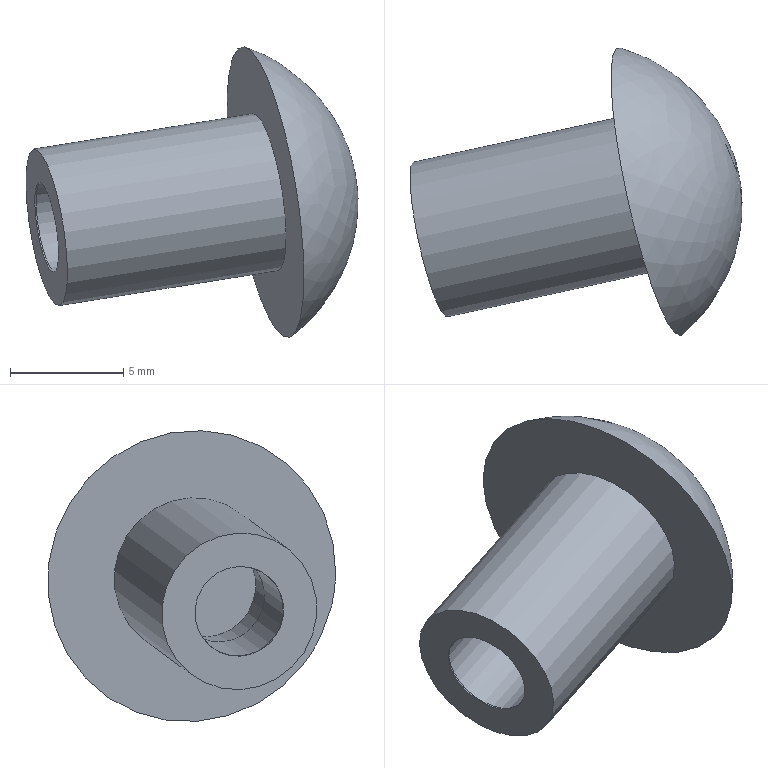Component | NX | 1_10 | 1 solid | 9 faces | box 14.65 x 12.71 x 12.84 mm | volume 581 mm3 | plane 4 | cylinder 3 | cone 1 | spline 1 | commonest cylinder face diameters 7 x1 4 x1 4.5 x1
STEP:
#1=CARTESIAN_POINT('',(0.,0.,0.));
#2=DIRECTION('',(0.,0.,1.));
#3=DIRECTION('',(1.,0.,0.));
#4=AXIS2_PLACEMENT_3D('',#1,#2,#3);
#5=CARTESIAN_POINT('',(119.694,214.706,-143.655));
#6=VERTEX_POINT('',#5);
#7=CARTESIAN_POINT('',(120.69,211.014,-144.855));
#8=VERTEX_POINT('',#7);
#9=CARTESIAN_POINT('',(120.192,212.86,-144.255));
#10=DIRECTION('',(0.9653,0.21,0.1554));
#11=DIRECTION('',(-0.2486,0.9212,0.2993));
#12=AXIS2_PLACEMENT_3D('',#9,#10,#11);
#13=CIRCLE('',#12,2.004);
#14=CARTESIAN_POINT('',(121.062,209.636,-145.303));
#15=DIRECTION('',(-0.9653,-0.21,-0.1554));
#16=DIRECTION('',(0.2486,-0.9212,-0.2993));
#17=AXIS2_PLACEMENT_3D('',#14,#15,#16);
#18=PLANE('',#17);
#19=CARTESIAN_POINT('',(-5.504,0.));
#20=CARTESIAN_POINT('',(-5.504,3.471));
#21=CARTESIAN_POINT('',(-2.498,1.735));
#22=CARTESIAN_POINT('',(0.5078,0.));
#23=CARTESIAN_POINT('',(-2.498,-1.735));
#24=CARTESIAN_POINT('',(-5.504,-3.471));
#25=CARTESIAN_POINT('',(-5.504,0.));
#26=(BOUNDED_CURVE()B_SPLINE_CURVE(2,(#19,#20,#21,#22,#23,#24,#25),.UNSPECIFIED.,.T.,.F.)B_SPLINE_CURVE_WITH_KNOTS((1,2,2,2,2,1),(-2.094,0.,2.094,4.189,6.283,8.378),.UNSPECIFIED.)CURVE()GEOMETRIC_REPRESENTATION_ITEM()RATIONAL_B_SPLINE_CURVE((1.,0.5,1.,0.5,1.,0.5,1.))REPRESENTATION_ITEM(''));
#27=(GEOMETRIC_REPRESENTATION_CONTEXT(2)PARAMETRIC_REPRESENTATION_CONTEXT()REPRESENTATION_CONTEXT('',''));
#28=DEFINITIONAL_REPRESENTATION('',(#26),#27);
#29=PCURVE('',#18,#28);
#30=CARTESIAN_POINT('',(120.192,212.86,-144.255));
#31=DIRECTION('',(-0.9653,-0.21,-0.1554));
#32=DIRECTION('',(0.2486,-0.9212,-0.2993));
#33=AXIS2_PLACEMENT_3D('',#30,#31,#32);
#34=CONICAL_SURFACE('',#33,2.004,0.0629);
#35=CARTESIAN_POINT('',(3.142,0.));
#36=DIRECTION('',(-1.,0.));
#37=VECTOR('',#36,1.);
#38=LINE('',#35,#37);
#39=(GEOMETRIC_REPRESENTATION_CONTEXT(2)PARAMETRIC_REPRESENTATION_CONTEXT()REPRESENTATION_CONTEXT('',''));
#40=DEFINITIONAL_REPRESENTATION('',(#38),#39);
#41=PCURVE('',#34,#40);
#42=SURFACE_CURVE('',#13,(#29,#41),.PCURVE_S1.);
#43=EDGE_CURVE('',#6,#8,#42,.T.);
#44=ORIENTED_EDGE('',*,*,#43,.T.);
#45=CARTESIAN_POINT('',(120.192,212.86,-144.255));
#46=DIRECTION('',(0.9653,0.21,0.1554));
#47=DIRECTION('',(-0.2486,0.9212,0.2993));
#48=AXIS2_PLACEMENT_3D('',#45,#46,#47);
#49=CIRCLE('',#48,2.004);
#50=CARTESIAN_POINT('',(-5.504,0.));
#51=CARTESIAN_POINT('',(-5.504,3.471));
#52=CARTESIAN_POINT('',(-2.498,1.735));
#53=CARTESIAN_POINT('',(0.5078,0.));
#54=CARTESIAN_POINT('',(-2.498,-1.735));
#55=CARTESIAN_POINT('',(-5.504,-3.471));
#56=CARTESIAN_POINT('',(-5.504,0.));
#57=(BOUNDED_CURVE()B_SPLINE_CURVE(2,(#50,#51,#52,#53,#54,#55,#56),.UNSPECIFIED.,.T.,.F.)B_SPLINE_CURVE_WITH_KNOTS((1,2,2,2,2,1),(-2.094,0.,2.094,4.189,6.283,8.378),.UNSPECIFIED.)CURVE()GEOMETRIC_REPRESENTATION_ITEM()RATIONAL_B_SPLINE_CURVE((1.,0.5,1.,0.5,1.,0.5,1.))REPRESENTATION_ITEM(''));
#58=(GEOMETRIC_REPRESENTATION_CONTEXT(2)PARAMETRIC_REPRESENTATION_CONTEXT()REPRESENTATION_CONTEXT('',''));
#59=DEFINITIONAL_REPRESENTATION('',(#57),#58);
#60=PCURVE('',#18,#59);
#61=CARTESIAN_POINT('',(9.425,0.));
#62=DIRECTION('',(-1.,0.));
#63=VECTOR('',#62,1.);
#64=LINE('',#61,#63);
#65=(GEOMETRIC_REPRESENTATION_CONTEXT(2)PARAMETRIC_REPRESENTATION_CONTEXT()REPRESENTATION_CONTEXT('',''));
#66=DEFINITIONAL_REPRESENTATION('',(#64),#65);
#67=PCURVE('',#34,#66);
#68=SURFACE_CURVE('',#49,(#60,#67),.PCURVE_S1.);
#69=EDGE_CURVE('',#8,#6,#68,.T.);
#70=ORIENTED_EDGE('',*,*,#69,.T.);
#71=EDGE_LOOP('',(#44,#70));
#72=FACE_BOUND('',#71,.T.);
#73=CARTESIAN_POINT('',(119.322,216.084,-143.208));
#74=VERTEX_POINT('',#73);
#75=CARTESIAN_POINT('',(120.192,212.86,-144.255));
#76=DIRECTION('',(0.9653,0.21,0.1554));
#77=DIRECTION('',(-0.2486,0.9212,0.2993));
#78=AXIS2_PLACEMENT_3D('',#75,#76,#77);
#79=CIRCLE('',#78,3.5);
#80=CARTESIAN_POINT('',(-7.,0.));
#81=CARTESIAN_POINT('',(-7.,6.062));
#82=CARTESIAN_POINT('',(-1.75,3.031));
#83=CARTESIAN_POINT('',(3.5,0.));
#84=CARTESIAN_POINT('',(-1.75,-3.031));
#85=CARTESIAN_POINT('',(-7.,-6.062));
#86=CARTESIAN_POINT('',(-7.,0.));
#87=(BOUNDED_CURVE()B_SPLINE_CURVE(2,(#80,#81,#82,#83,#84,#85,#86),.UNSPECIFIED.,.T.,.F.)B_SPLINE_CURVE_WITH_KNOTS((1,2,2,2,2,1),(-2.094,0.,2.094,4.189,6.283,8.378),.UNSPECIFIED.)CURVE()GEOMETRIC_REPRESENTATION_ITEM()RATIONAL_B_SPLINE_CURVE((1.,0.5,1.,0.5,1.,0.5,1.))REPRESENTATION_ITEM(''));
#88=(GEOMETRIC_REPRESENTATION_CONTEXT(2)PARAMETRIC_REPRESENTATION_CONTEXT()REPRESENTATION_CONTEXT('',''));
#89=DEFINITIONAL_REPRESENTATION('',(#87),#88);
#90=PCURVE('',#18,#89);
#91=CARTESIAN_POINT('',(129.845,214.96,-142.701));
#92=DIRECTION('',(0.9653,0.21,0.1554));
#93=DIRECTION('',(-0.2486,0.9212,0.2993));
#94=AXIS2_PLACEMENT_3D('',#91,#92,#93);
#95=CYLINDRICAL_SURFACE('',#94,3.5);
#96=CARTESIAN_POINT('',(0.,-10.));
#97=DIRECTION('',(1.,0.));
#98=VECTOR('',#97,1.);
#99=LINE('',#96,#98);
#100=(GEOMETRIC_REPRESENTATION_CONTEXT(2)PARAMETRIC_REPRESENTATION_CONTEXT()REPRESENTATION_CONTEXT('',''));
#101=DEFINITIONAL_REPRESENTATION('',(#99),#100);
#102=PCURVE('',#95,#101);
#103=SURFACE_CURVE('',#79,(#90,#102),.PCURVE_S1.);
#104=EDGE_CURVE('',#74,#74,#103,.T.);
#105=ORIENTED_EDGE('',*,*,#104,.F.);
#106=EDGE_LOOP('',(#105));
#107=FACE_BOUND('',#106,.T.);
#108=ADVANCED_FACE('',(#72,#107),#18,.T.);
#109=CARTESIAN_POINT('',(120.749,211.03,-144.844));
#110=VERTEX_POINT('',#109);
#111=CARTESIAN_POINT('',(120.252,212.873,-144.246));
#112=DIRECTION('',(-0.9653,-0.21,-0.1554));
#113=DIRECTION('',(0.2486,-0.9212,-0.2993));
#114=AXIS2_PLACEMENT_3D('',#111,#112,#113);
#115=CIRCLE('',#114,2.);
#116=CARTESIAN_POINT('',(0.,-0.06178));
#117=DIRECTION('',(1.,0.));
#118=VECTOR('',#117,1.);
#119=LINE('',#116,#118);
#120=(GEOMETRIC_REPRESENTATION_CONTEXT(2)PARAMETRIC_REPRESENTATION_CONTEXT()REPRESENTATION_CONTEXT('',''));
#121=DEFINITIONAL_REPRESENTATION('',(#119),#120);
#122=PCURVE('',#34,#121);
#123=CARTESIAN_POINT('',(124.053,213.7,-143.633));
#124=DIRECTION('',(-0.9653,-0.21,-0.1554));
#125=DIRECTION('',(0.2486,-0.9212,-0.2993));
#126=AXIS2_PLACEMENT_3D('',#123,#124,#125);
#127=CYLINDRICAL_SURFACE('',#126,2.);
#128=CARTESIAN_POINT('',(0.,3.938));
#129=DIRECTION('',(1.,0.));
#130=VECTOR('',#129,1.);
#131=LINE('',#128,#130);
#132=(GEOMETRIC_REPRESENTATION_CONTEXT(2)PARAMETRIC_REPRESENTATION_CONTEXT()REPRESENTATION_CONTEXT('',''));
#133=DEFINITIONAL_REPRESENTATION('',(#131),#132);
#134=PCURVE('',#127,#133);
#135=SURFACE_CURVE('',#115,(#122,#134),.PCURVE_S1.);
#136=EDGE_CURVE('',#110,#110,#135,.T.);
#137=ORIENTED_EDGE('',*,*,#136,.T.);
#138=CARTESIAN_POINT('',(120.749,211.03,-144.844));
#139=CARTESIAN_POINT('',(120.69,211.014,-144.855));
#140=B_SPLINE_CURVE_WITH_KNOTS('',1,(#138,#139),.UNSPECIFIED.,.F.,.F.,(2,2),(-0.0619,0.),.PIECEWISE_BEZIER_KNOTS.);
#141=CARTESIAN_POINT('',(6.283,0.));
#142=DIRECTION('',(0.,1.));
#143=VECTOR('',#142,1.);
#144=LINE('',#141,#143);
#145=(GEOMETRIC_REPRESENTATION_CONTEXT(2)PARAMETRIC_REPRESENTATION_CONTEXT()REPRESENTATION_CONTEXT('',''));
#146=DEFINITIONAL_REPRESENTATION('',(#144),#145);
#147=PCURVE('',#34,#146);
#148=CARTESIAN_POINT('',(0.,0.));
#149=DIRECTION('',(0.,1.));
#150=VECTOR('',#149,1.);
#151=LINE('',#148,#150);
#152=(GEOMETRIC_REPRESENTATION_CONTEXT(2)PARAMETRIC_REPRESENTATION_CONTEXT()REPRESENTATION_CONTEXT('',''));
#153=DEFINITIONAL_REPRESENTATION('',(#151),#152);
#154=PCURVE('',#34,#153);
#155=SEAM_CURVE('',#140,(#147,#154),.PCURVE_S1.);
#156=EDGE_CURVE('',#110,#8,#155,.T.);
#157=ORIENTED_EDGE('',*,*,#156,.T.);
#158=ORIENTED_EDGE('',*,*,#69,.T.);
#159=ORIENTED_EDGE('',*,*,#43,.T.);
#160=ORIENTED_EDGE('',*,*,#156,.F.);
#161=EDGE_LOOP('',(#137,#157,#158,#159,#160));
#162=FACE_BOUND('',#161,.F.);
#163=ADVANCED_FACE('',(#162),#34,.F.);
#164=CARTESIAN_POINT('',(128.229,220.948,-140.755));
#165=VERTEX_POINT('',#164);
#166=CARTESIAN_POINT('',(129.845,214.96,-142.701));
#167=DIRECTION('',(0.9653,0.21,0.1554));
#168=DIRECTION('',(-0.2486,0.9212,0.2993));
#169=AXIS2_PLACEMENT_3D('',#166,#167,#168);
#170=CIRCLE('',#169,6.5);
#171=CARTESIAN_POINT('',(133.706,215.8,-142.079));
#172=CARTESIAN_POINT('',(133.706,215.8,-142.079));
#173=CARTESIAN_POINT('',(133.706,215.8,-142.079));
#174=CARTESIAN_POINT('',(133.706,215.8,-142.079));
#175=CARTESIAN_POINT('',(133.706,215.8,-142.079));
#176=CARTESIAN_POINT('',(133.706,215.8,-142.079));
#177=CARTESIAN_POINT('',(133.706,215.8,-142.079));
#178=CARTESIAN_POINT('',(132.96,218.372,-141.248));
#179=CARTESIAN_POINT('',(132.51,216.535,-135.969));
#180=CARTESIAN_POINT('',(133.904,211.37,-137.647));
#181=CARTESIAN_POINT('',(134.354,213.207,-142.926));
#182=CARTESIAN_POINT('',(134.805,215.043,-148.205));
#183=CARTESIAN_POINT('',(133.411,220.209,-146.527));
#184=CARTESIAN_POINT('',(132.96,218.372,-141.248));
#185=CARTESIAN_POINT('',(130.948,220.263,-140.761));
#186=CARTESIAN_POINT('',(130.114,216.862,-130.986));
#187=CARTESIAN_POINT('',(132.695,207.297,-134.094));
#188=CARTESIAN_POINT('',(133.53,210.698,-143.869));
#189=CARTESIAN_POINT('',(134.364,214.099,-153.645));
#190=CARTESIAN_POINT('',(131.782,223.665,-150.537));
#191=CARTESIAN_POINT('',(130.948,220.263,-140.761));
#192=CARTESIAN_POINT('',(128.229,220.948,-140.755));
#193=CARTESIAN_POINT('',(127.184,216.689,-128.517));
#194=CARTESIAN_POINT('',(130.416,204.714,-132.408));
#195=CARTESIAN_POINT('',(131.461,208.972,-144.646));
#196=CARTESIAN_POINT('',(132.505,213.23,-156.885));
#197=CARTESIAN_POINT('',(129.273,225.206,-152.994));
#198=CARTESIAN_POINT('',(128.229,220.948,-140.755));
#199=(BOUNDED_SURFACE()B_SPLINE_SURFACE(3,3,((#171,#172,#173,#174,#175,#176,#177),(#178,#179,#180,#181,#182,#183,#184),(#185,#186,#187,#188,#189,#190,#191),(#192,#193,#194,#195,#196,#197,#198)),.UNSPECIFIED.,.F.,.T.,.F.)B_SPLINE_SURFACE_WITH_KNOTS((4,4),(1,3,3,3,1),(0.,1.),(-0.5,0.,0.5,1.,1.5),.UNSPECIFIED.)GEOMETRIC_REPRESENTATION_ITEM()RATIONAL_B_SPLINE_SURFACE(((1.,0.3333,0.3333,1.,0.3333,0.3333,1.),(0.9073,0.3024,0.3024,0.9073,0.3024,0.3024,0.9073),(0.9073,0.3024,0.3024,0.9073,0.3024,0.3024,0.9073),(1.,0.3333,0.3333,1.,0.3333,0.3333,1.)))REPRESENTATION_ITEM('')SURFACE());
#200=CARTESIAN_POINT('',(1.,0.));
#201=CARTESIAN_POINT('',(1.,0.02352));
#202=CARTESIAN_POINT('',(1.,0.06491));
#203=CARTESIAN_POINT('',(1.,0.1146));
#204=CARTESIAN_POINT('',(1.,0.1575));
#205=CARTESIAN_POINT('',(1.,0.196));
#206=CARTESIAN_POINT('',(1.,0.2322));
#207=CARTESIAN_POINT('',(1.,0.2678));
#208=CARTESIAN_POINT('',(1.,0.304));
#209=CARTESIAN_POINT('',(1.,0.3425));
#210=CARTESIAN_POINT('',(1.,0.3856));
#211=CARTESIAN_POINT('',(1.,0.4343));
#212=CARTESIAN_POINT('',(1.,0.5));
#213=CARTESIAN_POINT('',(1.,0.5657));
#214=CARTESIAN_POINT('',(1.,0.6144));
#215=CARTESIAN_POINT('',(1.,0.6575));
#216=CARTESIAN_POINT('',(1.,0.696));
#217=CARTESIAN_POINT('',(1.,0.7322));
#218=CARTESIAN_POINT('',(1.,0.7678));
#219=CARTESIAN_POINT('',(1.,0.804));
#220=CARTESIAN_POINT('',(1.,0.8425));
#221=CARTESIAN_POINT('',(1.,0.8854));
#222=CARTESIAN_POINT('',(1.,0.9351));
#223=CARTESIAN_POINT('',(1.,0.9765));
#224=CARTESIAN_POINT('',(1.,1.));
#225=B_SPLINE_CURVE_WITH_KNOTS('',3,(#200,#201,#202,#203,#204,#205,#206,#207,#208,#209,#210,#211,#212,#213,#214,#215,#216,#217,#218,#219,#220,#221,#222,#223,#224),.UNSPECIFIED.,.F.,.F.,(4,1,1,1,1,1,1,1,1,1,1,1,1,1,1,1,1,1,1,1,1,1,4),(0.,0.2856,0.5712,0.8568,1.142,1.428,1.714,1.999,2.285,2.57,2.856,3.142,3.427,3.713,3.998,4.284,4.57,4.855,5.141,5.426,5.712,5.998,6.283),.QUASI_UNIFORM_KNOTS.);
#226=(GEOMETRIC_REPRESENTATION_CONTEXT(2)PARAMETRIC_REPRESENTATION_CONTEXT()REPRESENTATION_CONTEXT('',''));
#227=DEFINITIONAL_REPRESENTATION('',(#225),#226);
#228=PCURVE('',#199,#227);
#229=CARTESIAN_POINT('',(131.461,208.972,-144.646));
#230=DIRECTION('',(-0.9653,-0.21,-0.1554));
#231=DIRECTION('',(0.2486,-0.9212,-0.2993));
#232=AXIS2_PLACEMENT_3D('',#229,#230,#231);
#233=PLANE('',#232);
#234=CARTESIAN_POINT('',(-13.,-0.));
#235=CARTESIAN_POINT('',(-13.,11.258));
#236=CARTESIAN_POINT('',(-3.25,5.629));
#237=CARTESIAN_POINT('',(6.5,-0.));
#238=CARTESIAN_POINT('',(-3.25,-5.629));
#239=CARTESIAN_POINT('',(-13.,-11.258));
#240=CARTESIAN_POINT('',(-13.,-0.));
#241=(BOUNDED_CURVE()B_SPLINE_CURVE(2,(#234,#235,#236,#237,#238,#239,#240),.UNSPECIFIED.,.T.,.F.)B_SPLINE_CURVE_WITH_KNOTS((1,2,2,2,2,1),(-2.094,0.,2.094,4.189,6.283,8.378),.UNSPECIFIED.)CURVE()GEOMETRIC_REPRESENTATION_ITEM()RATIONAL_B_SPLINE_CURVE((1.,0.5,1.,0.5,1.,0.5,1.))REPRESENTATION_ITEM(''));
#242=(GEOMETRIC_REPRESENTATION_CONTEXT(2)PARAMETRIC_REPRESENTATION_CONTEXT()REPRESENTATION_CONTEXT('',''));
#243=DEFINITIONAL_REPRESENTATION('',(#241),#242);
#244=PCURVE('',#233,#243);
#245=SURFACE_CURVE('',#170,(#228,#244),.PCURVE_S1.);
#246=EDGE_CURVE('',#165,#165,#245,.T.);
#247=ORIENTED_EDGE('',*,*,#246,.T.);
#248=CARTESIAN_POINT('',(133.706,215.8,-142.079));
#249=VERTEX_POINT('',#248);
#250=CARTESIAN_POINT('',(133.706,215.8,-142.079));
#251=CARTESIAN_POINT('',(132.96,218.372,-141.248));
#252=CARTESIAN_POINT('',(130.948,220.263,-140.761));
#253=CARTESIAN_POINT('',(128.229,220.948,-140.755));
#254=(BOUNDED_CURVE()B_SPLINE_CURVE(3,(#250,#251,#252,#253),.UNSPECIFIED.,.F.,.F.)B_SPLINE_CURVE_WITH_KNOTS((4,4),(0.,1.),.PIECEWISE_BEZIER_KNOTS.)CURVE()GEOMETRIC_REPRESENTATION_ITEM()RATIONAL_B_SPLINE_CURVE((1.,0.9073,0.9073,1.))REPRESENTATION_ITEM(''));
#255=CARTESIAN_POINT('',(0.,1.));
#256=DIRECTION('',(1.,0.));
#257=VECTOR('',#256,1.);
#258=LINE('',#255,#257);
#259=(GEOMETRIC_REPRESENTATION_CONTEXT(2)PARAMETRIC_REPRESENTATION_CONTEXT()REPRESENTATION_CONTEXT('',''));
#260=DEFINITIONAL_REPRESENTATION('',(#258),#259);
#261=PCURVE('',#199,#260);
#262=CARTESIAN_POINT('',(0.,0.));
#263=DIRECTION('',(1.,0.));
#264=VECTOR('',#263,1.);
#265=LINE('',#262,#264);
#266=(GEOMETRIC_REPRESENTATION_CONTEXT(2)PARAMETRIC_REPRESENTATION_CONTEXT()REPRESENTATION_CONTEXT('',''));
#267=DEFINITIONAL_REPRESENTATION('',(#265),#266);
#268=PCURVE('',#199,#267);
#269=SEAM_CURVE('',#254,(#261,#268),.PCURVE_S1.);
#270=EDGE_CURVE('',#249,#165,#269,.T.);
#271=ORIENTED_EDGE('',*,*,#270,.F.);
#272=ORIENTED_EDGE('',*,*,#270,.T.);
#273=EDGE_LOOP('',(#247,#271,#272));
#274=FACE_BOUND('',#273,.T.);
#275=ADVANCED_FACE('',(#274),#199,.T.);
#276=CARTESIAN_POINT('',(128.975,218.184,-141.653));
#277=VERTEX_POINT('',#276);
#278=CARTESIAN_POINT('',(129.845,214.96,-142.701));
#279=DIRECTION('',(0.9653,0.21,0.1554));
#280=DIRECTION('',(-0.2486,0.9212,0.2993));
#281=AXIS2_PLACEMENT_3D('',#278,#279,#280);
#282=CIRCLE('',#281,3.5);
#283=CARTESIAN_POINT('',(-10.,-0.));
#284=CARTESIAN_POINT('',(-10.,6.062));
#285=CARTESIAN_POINT('',(-4.75,3.031));
#286=CARTESIAN_POINT('',(0.5,-0.));
#287=CARTESIAN_POINT('',(-4.75,-3.031));
#288=CARTESIAN_POINT('',(-10.,-6.062));
#289=CARTESIAN_POINT('',(-10.,-0.));
#290=(BOUNDED_CURVE()B_SPLINE_CURVE(2,(#283,#284,#285,#286,#287,#288,#289),.UNSPECIFIED.,.T.,.F.)B_SPLINE_CURVE_WITH_KNOTS((1,2,2,2,2,1),(-2.094,0.,2.094,4.189,6.283,8.378),.UNSPECIFIED.)CURVE()GEOMETRIC_REPRESENTATION_ITEM()RATIONAL_B_SPLINE_CURVE((1.,0.5,1.,0.5,1.,0.5,1.))REPRESENTATION_ITEM(''));
#291=(GEOMETRIC_REPRESENTATION_CONTEXT(2)PARAMETRIC_REPRESENTATION_CONTEXT()REPRESENTATION_CONTEXT('',''));
#292=DEFINITIONAL_REPRESENTATION('',(#290),#291);
#293=PCURVE('',#233,#292);
#294=CARTESIAN_POINT('',(0.,0.));
#295=DIRECTION('',(1.,0.));
#296=VECTOR('',#295,1.);
#297=LINE('',#294,#296);
#298=(GEOMETRIC_REPRESENTATION_CONTEXT(2)PARAMETRIC_REPRESENTATION_CONTEXT()REPRESENTATION_CONTEXT('',''));
#299=DEFINITIONAL_REPRESENTATION('',(#297),#298);
#300=PCURVE('',#95,#299);
#301=SURFACE_CURVE('',#282,(#293,#300),.PCURVE_S1.);
#302=EDGE_CURVE('',#277,#277,#301,.T.);
#303=ORIENTED_EDGE('',*,*,#302,.T.);
#304=EDGE_LOOP('',(#303));
#305=FACE_BOUND('',#304,.T.);
#306=ORIENTED_EDGE('',*,*,#246,.F.);
#307=EDGE_LOOP('',(#306));
#308=FACE_BOUND('',#307,.T.);
#309=ADVANCED_FACE('',(#305,#308),#233,.T.);
#310=ORIENTED_EDGE('',*,*,#104,.T.);
#311=CARTESIAN_POINT('',(119.322,216.084,-143.208));
#312=CARTESIAN_POINT('',(128.975,218.184,-141.653));
#313=B_SPLINE_CURVE_WITH_KNOTS('',1,(#311,#312),.UNSPECIFIED.,.F.,.F.,(2,2),(-10.,0.),.PIECEWISE_BEZIER_KNOTS.);
#314=CARTESIAN_POINT('',(6.283,0.));
#315=DIRECTION('',(0.,1.));
#316=VECTOR('',#315,1.);
#317=LINE('',#314,#316);
#318=(GEOMETRIC_REPRESENTATION_CONTEXT(2)PARAMETRIC_REPRESENTATION_CONTEXT()REPRESENTATION_CONTEXT('',''));
#319=DEFINITIONAL_REPRESENTATION('',(#317),#318);
#320=PCURVE('',#95,#319);
#321=CARTESIAN_POINT('',(0.,0.));
#322=DIRECTION('',(0.,1.));
#323=VECTOR('',#322,1.);
#324=LINE('',#321,#323);
#325=(GEOMETRIC_REPRESENTATION_CONTEXT(2)PARAMETRIC_REPRESENTATION_CONTEXT()REPRESENTATION_CONTEXT('',''));
#326=DEFINITIONAL_REPRESENTATION('',(#324),#325);
#327=PCURVE('',#95,#326);
#328=SEAM_CURVE('',#313,(#320,#327),.PCURVE_S1.);
#329=EDGE_CURVE('',#74,#277,#328,.T.);
#330=ORIENTED_EDGE('',*,*,#329,.T.);
#331=ORIENTED_EDGE('',*,*,#302,.F.);
#332=ORIENTED_EDGE('',*,*,#329,.F.);
#333=EDGE_LOOP('',(#310,#330,#331,#332));
#334=FACE_BOUND('',#333,.T.);
#335=ADVANCED_FACE('',(#334),#95,.T.);
#336=ORIENTED_EDGE('',*,*,#136,.F.);
#337=CARTESIAN_POINT('',(124.55,211.857,-144.232));
#338=VERTEX_POINT('',#337);
#339=CARTESIAN_POINT('',(124.55,211.857,-144.232));
#340=CARTESIAN_POINT('',(120.749,211.03,-144.844));
#341=B_SPLINE_CURVE_WITH_KNOTS('',1,(#339,#340),.UNSPECIFIED.,.F.,.F.,(2,2),(0.,3.938),.PIECEWISE_BEZIER_KNOTS.);
#342=CARTESIAN_POINT('',(0.,0.));
#343=DIRECTION('',(0.,1.));
#344=VECTOR('',#343,1.);
#345=LINE('',#342,#344);
#346=(GEOMETRIC_REPRESENTATION_CONTEXT(2)PARAMETRIC_REPRESENTATION_CONTEXT()REPRESENTATION_CONTEXT('',''));
#347=DEFINITIONAL_REPRESENTATION('',(#345),#346);
#348=PCURVE('',#127,#347);
#349=CARTESIAN_POINT('',(6.283,0.));
#350=DIRECTION('',(0.,1.));
#351=VECTOR('',#350,1.);
#352=LINE('',#349,#351);
#353=(GEOMETRIC_REPRESENTATION_CONTEXT(2)PARAMETRIC_REPRESENTATION_CONTEXT()REPRESENTATION_CONTEXT('',''));
#354=DEFINITIONAL_REPRESENTATION('',(#352),#353);
#355=PCURVE('',#127,#354);
#356=SEAM_CURVE('',#341,(#348,#355),.PCURVE_S1.);
#357=EDGE_CURVE('',#338,#110,#356,.T.);
#358=ORIENTED_EDGE('',*,*,#357,.F.);
#359=CARTESIAN_POINT('',(124.053,213.7,-143.633));
#360=DIRECTION('',(-0.9653,-0.21,-0.1554));
#361=DIRECTION('',(0.2486,-0.9212,-0.2993));
#362=AXIS2_PLACEMENT_3D('',#359,#360,#361);
#363=CIRCLE('',#362,2.);
#364=CARTESIAN_POINT('',(0.,0.));
#365=DIRECTION('',(1.,0.));
#366=VECTOR('',#365,1.);
#367=LINE('',#364,#366);
#368=(GEOMETRIC_REPRESENTATION_CONTEXT(2)PARAMETRIC_REPRESENTATION_CONTEXT()REPRESENTATION_CONTEXT('',''));
#369=DEFINITIONAL_REPRESENTATION('',(#367),#368);
#370=PCURVE('',#127,#369);
#371=CARTESIAN_POINT('',(124.489,212.086,-144.158));
#372=DIRECTION('',(0.9653,0.21,0.1554));
#373=DIRECTION('',(-0.2486,0.9212,0.2993));
#374=AXIS2_PLACEMENT_3D('',#371,#372,#373);
#375=PLANE('',#374);
#376=CARTESIAN_POINT('',(-0.2481,0.));
#377=CARTESIAN_POINT('',(-0.2481,3.464));
#378=CARTESIAN_POINT('',(2.752,1.732));
#379=CARTESIAN_POINT('',(5.752,0.));
#380=CARTESIAN_POINT('',(2.752,-1.732));
#381=CARTESIAN_POINT('',(-0.2481,-3.464));
#382=CARTESIAN_POINT('',(-0.2481,0.));
#383=(BOUNDED_CURVE()B_SPLINE_CURVE(2,(#376,#377,#378,#379,#380,#381,#382),.UNSPECIFIED.,.T.,.F.)B_SPLINE_CURVE_WITH_KNOTS((1,2,2,2,2,1),(-2.094,0.,2.094,4.189,6.283,8.378),.UNSPECIFIED.)CURVE()GEOMETRIC_REPRESENTATION_ITEM()RATIONAL_B_SPLINE_CURVE((1.,0.5,1.,0.5,1.,0.5,1.))REPRESENTATION_ITEM(''));
#384=(GEOMETRIC_REPRESENTATION_CONTEXT(2)PARAMETRIC_REPRESENTATION_CONTEXT()REPRESENTATION_CONTEXT('',''));
#385=DEFINITIONAL_REPRESENTATION('',(#383),#384);
#386=PCURVE('',#375,#385);
#387=SURFACE_CURVE('',#363,(#370,#386),.PCURVE_S1.);
#388=EDGE_CURVE('',#338,#338,#387,.T.);
#389=ORIENTED_EDGE('',*,*,#388,.T.);
#390=ORIENTED_EDGE('',*,*,#357,.T.);
#391=EDGE_LOOP('',(#336,#358,#389,#390));
#392=FACE_BOUND('',#391,.F.);
#393=ADVANCED_FACE('',(#392),#127,.F.);
#394=CARTESIAN_POINT('',(127.508,212.257,-143.841));
#395=VERTEX_POINT('',#394);
#396=CARTESIAN_POINT('',(126.949,214.33,-143.167));
#397=DIRECTION('',(-0.9653,-0.21,-0.1554));
#398=DIRECTION('',(0.2486,-0.9212,-0.2993));
#399=AXIS2_PLACEMENT_3D('',#396,#397,#398);
#400=CIRCLE('',#399,2.25);
#401=CARTESIAN_POINT('',(127.446,212.487,-143.766));
#402=DIRECTION('',(-0.9653,-0.21,-0.1554));
#403=DIRECTION('',(0.2486,-0.9212,-0.2993));
#404=AXIS2_PLACEMENT_3D('',#401,#402,#403);
#405=PLANE('',#404);
#406=CARTESIAN_POINT('',(-2.,0.));
#407=DIRECTION('',(1.,0.));
#408=AXIS2_PLACEMENT_2D('',#406,#407);
#409=CIRCLE('',#408,2.25);
#410=(GEOMETRIC_REPRESENTATION_CONTEXT(2)PARAMETRIC_REPRESENTATION_CONTEXT()REPRESENTATION_CONTEXT('',''));
#411=DEFINITIONAL_REPRESENTATION('',(#409),#410);
#412=PCURVE('',#405,#411);
#413=CARTESIAN_POINT('',(126.949,214.33,-143.167));
#414=DIRECTION('',(-0.9653,-0.21,-0.1554));
#415=DIRECTION('',(0.2486,-0.9212,-0.2993));
#416=AXIS2_PLACEMENT_3D('',#413,#414,#415);
#417=CYLINDRICAL_SURFACE('',#416,2.25);
#418=CARTESIAN_POINT('',(0.,0.));
#419=DIRECTION('',(1.,0.));
#420=VECTOR('',#419,1.);
#421=LINE('',#418,#420);
#422=(GEOMETRIC_REPRESENTATION_CONTEXT(2)PARAMETRIC_REPRESENTATION_CONTEXT()REPRESENTATION_CONTEXT('',''));
#423=DEFINITIONAL_REPRESENTATION('',(#421),#422);
#424=PCURVE('',#417,#423);
#425=SURFACE_CURVE('',#400,(#412,#424),.PCURVE_S1.);
#426=EDGE_CURVE('',#395,#395,#425,.T.);
#427=ORIENTED_EDGE('',*,*,#426,.T.);
#428=EDGE_LOOP('',(#427));
#429=FACE_BOUND('',#428,.T.);
#430=ADVANCED_FACE('',(#429),#405,.T.);
#431=CARTESIAN_POINT('',(124.612,211.627,-144.307));
#432=VERTEX_POINT('',#431);
#433=CARTESIAN_POINT('',(124.053,213.7,-143.633));
#434=DIRECTION('',(0.9653,0.21,0.1554));
#435=DIRECTION('',(0.2486,-0.9212,-0.2993));
#436=AXIS2_PLACEMENT_3D('',#433,#434,#435);
#437=CIRCLE('',#436,2.25);
#438=CARTESIAN_POINT('',(6.283,3.));
#439=DIRECTION('',(-1.,0.));
#440=VECTOR('',#439,1.);
#441=LINE('',#438,#440);
#442=(GEOMETRIC_REPRESENTATION_CONTEXT(2)PARAMETRIC_REPRESENTATION_CONTEXT()REPRESENTATION_CONTEXT('',''));
#443=DEFINITIONAL_REPRESENTATION('',(#441),#442);
#444=PCURVE('',#417,#443);
#445=CARTESIAN_POINT('',(1.752,0.));
#446=DIRECTION('',(-1.,0.));
#447=AXIS2_PLACEMENT_2D('',#445,#446);
#448=CIRCLE('',#447,2.25);
#449=(GEOMETRIC_REPRESENTATION_CONTEXT(2)PARAMETRIC_REPRESENTATION_CONTEXT()REPRESENTATION_CONTEXT('',''));
#450=DEFINITIONAL_REPRESENTATION('',(#448),#449);
#451=PCURVE('',#375,#450);
#452=SURFACE_CURVE('',#437,(#444,#451),.PCURVE_S1.);
#453=EDGE_CURVE('',#432,#432,#452,.T.);
#454=ORIENTED_EDGE('',*,*,#453,.T.);
#455=CARTESIAN_POINT('',(127.508,212.257,-143.841));
#456=CARTESIAN_POINT('',(124.612,211.627,-144.307));
#457=B_SPLINE_CURVE_WITH_KNOTS('',1,(#455,#456),.UNSPECIFIED.,.F.,.F.,(2,2),(0.,3.),.PIECEWISE_BEZIER_KNOTS.);
#458=CARTESIAN_POINT('',(0.,0.));
#459=DIRECTION('',(0.,1.));
#460=VECTOR('',#459,1.);
#461=LINE('',#458,#460);
#462=(GEOMETRIC_REPRESENTATION_CONTEXT(2)PARAMETRIC_REPRESENTATION_CONTEXT()REPRESENTATION_CONTEXT('',''));
#463=DEFINITIONAL_REPRESENTATION('',(#461),#462);
#464=PCURVE('',#417,#463);
#465=CARTESIAN_POINT('',(6.283,0.));
#466=DIRECTION('',(0.,1.));
#467=VECTOR('',#466,1.);
#468=LINE('',#465,#467);
#469=(GEOMETRIC_REPRESENTATION_CONTEXT(2)PARAMETRIC_REPRESENTATION_CONTEXT()REPRESENTATION_CONTEXT('',''));
#470=DEFINITIONAL_REPRESENTATION('',(#468),#469);
#471=PCURVE('',#417,#470);
#472=SEAM_CURVE('',#457,(#464,#471),.PCURVE_S1.);
#473=EDGE_CURVE('',#395,#432,#472,.T.);
#474=ORIENTED_EDGE('',*,*,#473,.F.);
#475=ORIENTED_EDGE('',*,*,#426,.T.);
#476=ORIENTED_EDGE('',*,*,#473,.T.);
#477=EDGE_LOOP('',(#454,#474,#475,#476));
#478=FACE_BOUND('',#477,.F.);
#479=ADVANCED_FACE('',(#478),#417,.F.);
#480=ORIENTED_EDGE('',*,*,#388,.T.);
#481=EDGE_LOOP('',(#480));
#482=FACE_BOUND('',#481,.T.);
#483=ORIENTED_EDGE('',*,*,#453,.T.);
#484=EDGE_LOOP('',(#483));
#485=FACE_BOUND('',#484,.T.);
#486=ADVANCED_FACE('',(#482,#485),#375,.T.);
#487=CLOSED_SHELL('',(#108,#163,#275,#309,#335,#393,#430,#479,#486));
#488=MANIFOLD_SOLID_BREP('',#487);
#489=(LENGTH_UNIT()NAMED_UNIT(*)SI_UNIT(.MILLI.,.METRE.));
#490=UNCERTAINTY_MEASURE_WITH_UNIT(LENGTH_MEASURE(0.00001),#489,'','');
#491=(NAMED_UNIT(*)PLANE_ANGLE_UNIT()SI_UNIT($,.RADIAN.));
#492=(NAMED_UNIT(*)SI_UNIT($,.STERADIAN.)SOLID_ANGLE_UNIT());
#493=(GEOMETRIC_REPRESENTATION_CONTEXT(3)GLOBAL_UNCERTAINTY_ASSIGNED_CONTEXT((#490))GLOBAL_UNIT_ASSIGNED_CONTEXT((#489,#491,#492))REPRESENTATION_CONTEXT('',''));
#494=ADVANCED_BREP_SHAPE_REPRESENTATION('',(#4,#488),#493);